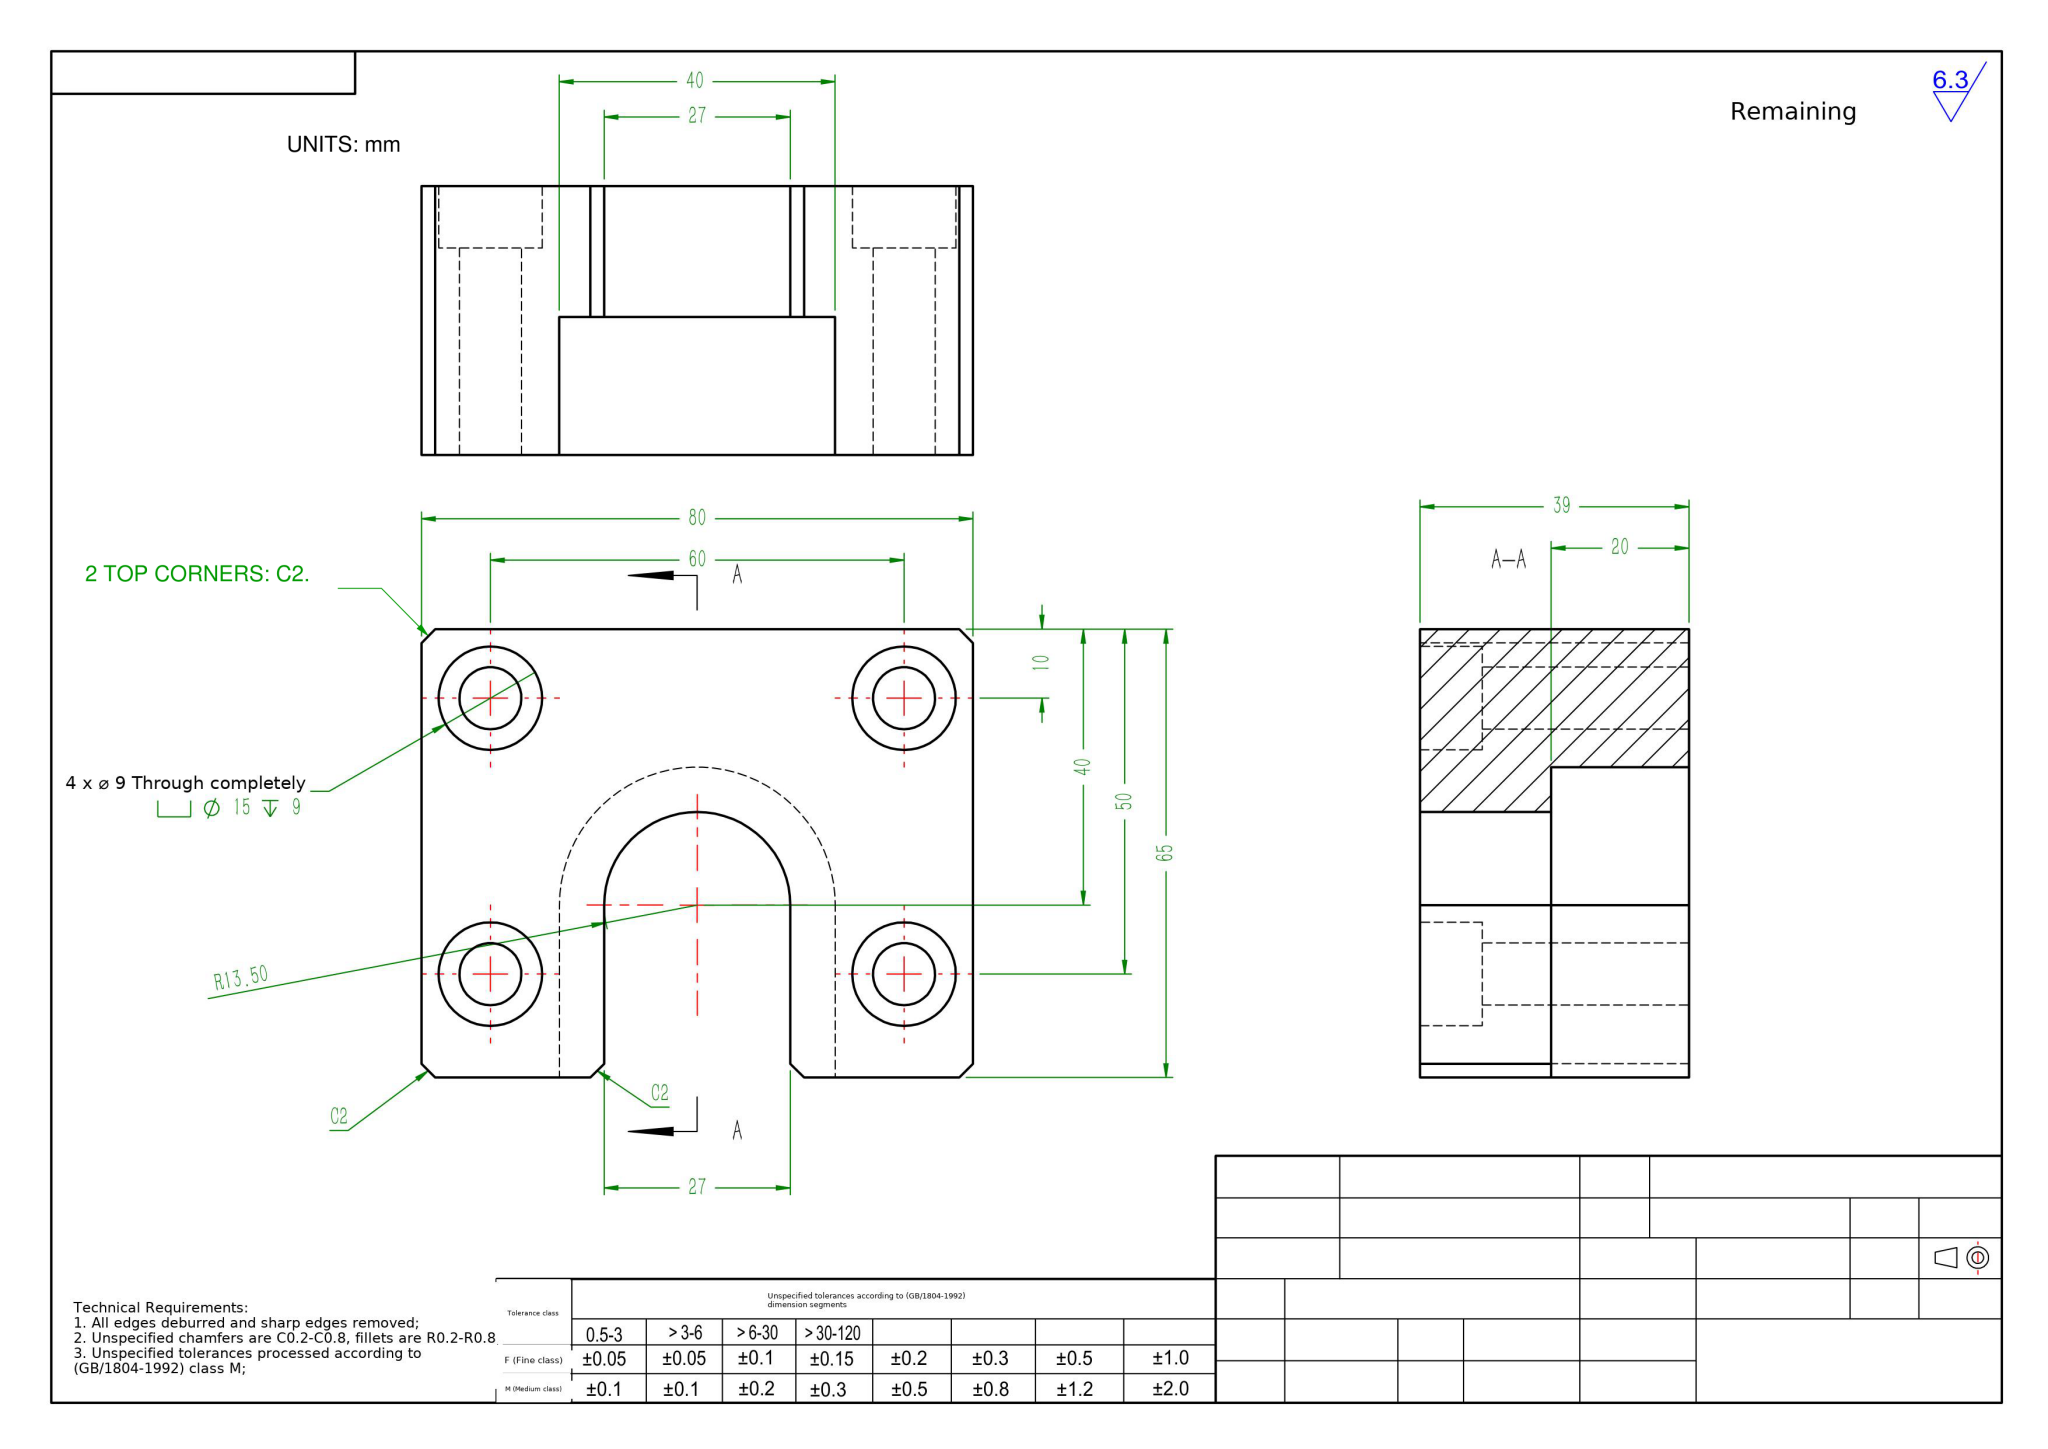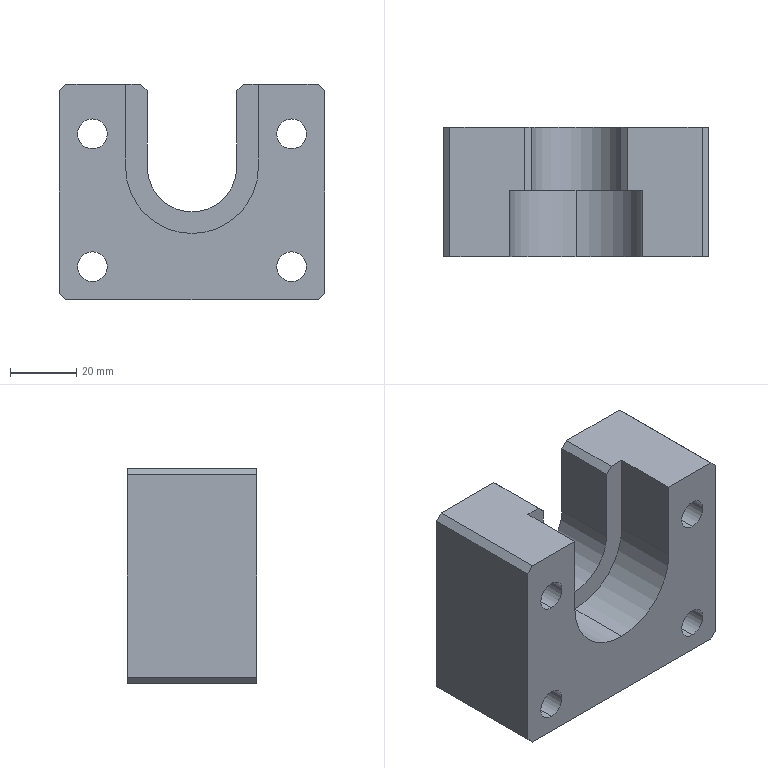Part | NX | mm | 1 solid | 41 faces | box 80 x 39 x 65 mm | volume 137586 mm3 | plane 22 | cylinder 19 | commonest cylinder face diameters 15 x8 9 x8 40 x2 27 x1